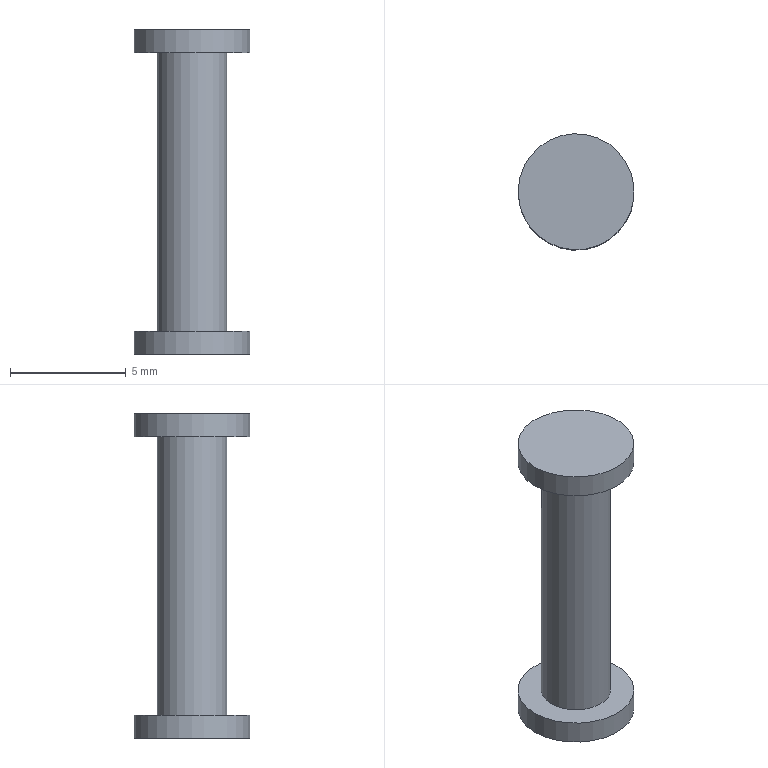Component | NX | PIN | 1 solid | 7 faces | box 5 x 5 x 14 mm | volume 124 mm3 | plane 4 | cylinder 3 | commonest cylinder face diameters 5 x2 3 x1
STEP:
#1=CARTESIAN_POINT('',(0.,0.,0.));
#2=DIRECTION('',(0.,0.,1.));
#3=DIRECTION('',(1.,0.,0.));
#4=AXIS2_PLACEMENT_3D('',#1,#2,#3);
#5=CARTESIAN_POINT('',(-11.268,-58.059,25.35));
#6=VERTEX_POINT('',#5);
#7=CARTESIAN_POINT('',(-9.005,-59.121,25.35));
#8=DIRECTION('',(0.,0.,1.));
#9=DIRECTION('',(-0.9054,0.4247,0.));
#10=AXIS2_PLACEMENT_3D('',#7,#8,#9);
#11=CIRCLE('',#10,2.5);
#12=CARTESIAN_POINT('',(-11.268,-58.059,25.35));
#13=DIRECTION('',(0.,0.,-1.));
#14=DIRECTION('',(0.9054,-0.4247,0.));
#15=AXIS2_PLACEMENT_3D('',#12,#13,#14);
#16=PLANE('',#15);
#17=CARTESIAN_POINT('',(0.,-0.));
#18=CARTESIAN_POINT('',(0.,4.33));
#19=CARTESIAN_POINT('',(3.75,2.165));
#20=CARTESIAN_POINT('',(7.5,-0.));
#21=CARTESIAN_POINT('',(3.75,-2.165));
#22=CARTESIAN_POINT('',(0.,-4.33));
#23=CARTESIAN_POINT('',(0.,-0.));
#24=(BOUNDED_CURVE()B_SPLINE_CURVE(2,(#17,#18,#19,#20,#21,#22,#23),.UNSPECIFIED.,.T.,.F.)B_SPLINE_CURVE_WITH_KNOTS((1,2,2,2,2,1),(-2.094,0.,2.094,4.189,6.283,8.378),.UNSPECIFIED.)CURVE()GEOMETRIC_REPRESENTATION_ITEM()RATIONAL_B_SPLINE_CURVE((1.,0.5,1.,0.5,1.,0.5,1.))REPRESENTATION_ITEM(''));
#25=(GEOMETRIC_REPRESENTATION_CONTEXT(2)PARAMETRIC_REPRESENTATION_CONTEXT()REPRESENTATION_CONTEXT('',''));
#26=DEFINITIONAL_REPRESENTATION('',(#24),#25);
#27=PCURVE('',#16,#26);
#28=CARTESIAN_POINT('',(-9.005,-59.121,25.35));
#29=DIRECTION('',(0.,0.,1.));
#30=DIRECTION('',(-0.9054,0.4247,0.));
#31=AXIS2_PLACEMENT_3D('',#28,#29,#30);
#32=CYLINDRICAL_SURFACE('',#31,2.5);
#33=CARTESIAN_POINT('',(0.,0.));
#34=DIRECTION('',(1.,0.));
#35=VECTOR('',#34,1.);
#36=LINE('',#33,#35);
#37=(GEOMETRIC_REPRESENTATION_CONTEXT(2)PARAMETRIC_REPRESENTATION_CONTEXT()REPRESENTATION_CONTEXT('',''));
#38=DEFINITIONAL_REPRESENTATION('',(#36),#37);
#39=PCURVE('',#32,#38);
#40=SURFACE_CURVE('',#11,(#27,#39),.PCURVE_S1.);
#41=EDGE_CURVE('',#6,#6,#40,.T.);
#42=ORIENTED_EDGE('',*,*,#41,.F.);
#43=EDGE_LOOP('',(#42));
#44=FACE_BOUND('',#43,.T.);
#45=ADVANCED_FACE('',(#44),#16,.T.);
#46=ORIENTED_EDGE('',*,*,#41,.T.);
#47=CARTESIAN_POINT('',(-11.268,-58.059,26.35));
#48=VERTEX_POINT('',#47);
#49=CARTESIAN_POINT('',(-11.268,-58.059,25.35));
#50=CARTESIAN_POINT('',(-11.268,-58.059,26.35));
#51=B_SPLINE_CURVE_WITH_KNOTS('',1,(#49,#50),.UNSPECIFIED.,.F.,.F.,(2,2),(0.,1.),.PIECEWISE_BEZIER_KNOTS.);
#52=CARTESIAN_POINT('',(6.283,0.));
#53=DIRECTION('',(0.,1.));
#54=VECTOR('',#53,1.);
#55=LINE('',#52,#54);
#56=(GEOMETRIC_REPRESENTATION_CONTEXT(2)PARAMETRIC_REPRESENTATION_CONTEXT()REPRESENTATION_CONTEXT('',''));
#57=DEFINITIONAL_REPRESENTATION('',(#55),#56);
#58=PCURVE('',#32,#57);
#59=CARTESIAN_POINT('',(0.,0.));
#60=DIRECTION('',(0.,1.));
#61=VECTOR('',#60,1.);
#62=LINE('',#59,#61);
#63=(GEOMETRIC_REPRESENTATION_CONTEXT(2)PARAMETRIC_REPRESENTATION_CONTEXT()REPRESENTATION_CONTEXT('',''));
#64=DEFINITIONAL_REPRESENTATION('',(#62),#63);
#65=PCURVE('',#32,#64);
#66=SEAM_CURVE('',#51,(#58,#65),.PCURVE_S1.);
#67=EDGE_CURVE('',#6,#48,#66,.T.);
#68=ORIENTED_EDGE('',*,*,#67,.T.);
#69=CARTESIAN_POINT('',(-9.005,-59.121,26.35));
#70=DIRECTION('',(0.,0.,1.));
#71=DIRECTION('',(-0.9054,0.4247,0.));
#72=AXIS2_PLACEMENT_3D('',#69,#70,#71);
#73=CIRCLE('',#72,2.5);
#74=CARTESIAN_POINT('',(0.,1.));
#75=DIRECTION('',(1.,0.));
#76=VECTOR('',#75,1.);
#77=LINE('',#74,#76);
#78=(GEOMETRIC_REPRESENTATION_CONTEXT(2)PARAMETRIC_REPRESENTATION_CONTEXT()REPRESENTATION_CONTEXT('',''));
#79=DEFINITIONAL_REPRESENTATION('',(#77),#78);
#80=PCURVE('',#32,#79);
#81=CARTESIAN_POINT('',(-10.363,-58.484,26.35));
#82=DIRECTION('',(0.,0.,1.));
#83=DIRECTION('',(-0.9054,0.4247,0.));
#84=AXIS2_PLACEMENT_3D('',#81,#82,#83);
#85=PLANE('',#84);
#86=CARTESIAN_POINT('',(-1.5,0.));
#87=DIRECTION('',(1.,0.));
#88=AXIS2_PLACEMENT_2D('',#86,#87);
#89=CIRCLE('',#88,2.5);
#90=(GEOMETRIC_REPRESENTATION_CONTEXT(2)PARAMETRIC_REPRESENTATION_CONTEXT()REPRESENTATION_CONTEXT('',''));
#91=DEFINITIONAL_REPRESENTATION('',(#89),#90);
#92=PCURVE('',#85,#91);
#93=SURFACE_CURVE('',#73,(#80,#92),.PCURVE_S1.);
#94=EDGE_CURVE('',#48,#48,#93,.T.);
#95=ORIENTED_EDGE('',*,*,#94,.F.);
#96=ORIENTED_EDGE('',*,*,#67,.F.);
#97=EDGE_LOOP('',(#46,#68,#95,#96));
#98=FACE_BOUND('',#97,.T.);
#99=ADVANCED_FACE('',(#98),#32,.T.);
#100=ORIENTED_EDGE('',*,*,#94,.T.);
#101=EDGE_LOOP('',(#100));
#102=FACE_BOUND('',#101,.T.);
#103=CARTESIAN_POINT('',(-10.363,-58.484,26.35));
#104=VERTEX_POINT('',#103);
#105=CARTESIAN_POINT('',(-9.005,-59.121,26.35));
#106=DIRECTION('',(0.,0.,1.));
#107=DIRECTION('',(-0.9054,0.4247,0.));
#108=AXIS2_PLACEMENT_3D('',#105,#106,#107);
#109=CIRCLE('',#108,1.5);
#110=CARTESIAN_POINT('',(-1.5,0.));
#111=DIRECTION('',(1.,0.));
#112=AXIS2_PLACEMENT_2D('',#110,#111);
#113=CIRCLE('',#112,1.5);
#114=(GEOMETRIC_REPRESENTATION_CONTEXT(2)PARAMETRIC_REPRESENTATION_CONTEXT()REPRESENTATION_CONTEXT('',''));
#115=DEFINITIONAL_REPRESENTATION('',(#113),#114);
#116=PCURVE('',#85,#115);
#117=CARTESIAN_POINT('',(-9.005,-59.121,25.35));
#118=DIRECTION('',(0.,0.,1.));
#119=DIRECTION('',(-0.9054,0.4247,0.));
#120=AXIS2_PLACEMENT_3D('',#117,#118,#119);
#121=CYLINDRICAL_SURFACE('',#120,1.5);
#122=CARTESIAN_POINT('',(0.,1.));
#123=DIRECTION('',(1.,0.));
#124=VECTOR('',#123,1.);
#125=LINE('',#122,#124);
#126=(GEOMETRIC_REPRESENTATION_CONTEXT(2)PARAMETRIC_REPRESENTATION_CONTEXT()REPRESENTATION_CONTEXT('',''));
#127=DEFINITIONAL_REPRESENTATION('',(#125),#126);
#128=PCURVE('',#121,#127);
#129=SURFACE_CURVE('',#109,(#116,#128),.PCURVE_S1.);
#130=EDGE_CURVE('',#104,#104,#129,.T.);
#131=ORIENTED_EDGE('',*,*,#130,.F.);
#132=EDGE_LOOP('',(#131));
#133=FACE_BOUND('',#132,.T.);
#134=ADVANCED_FACE('',(#102,#133),#85,.T.);
#135=ORIENTED_EDGE('',*,*,#130,.T.);
#136=CARTESIAN_POINT('',(-10.363,-58.484,38.35));
#137=VERTEX_POINT('',#136);
#138=CARTESIAN_POINT('',(-10.363,-58.484,26.35));
#139=CARTESIAN_POINT('',(-10.363,-58.484,38.35));
#140=B_SPLINE_CURVE_WITH_KNOTS('',1,(#138,#139),.UNSPECIFIED.,.F.,.F.,(2,2),(1.,13.),.PIECEWISE_BEZIER_KNOTS.);
#141=CARTESIAN_POINT('',(6.283,0.));
#142=DIRECTION('',(0.,1.));
#143=VECTOR('',#142,1.);
#144=LINE('',#141,#143);
#145=(GEOMETRIC_REPRESENTATION_CONTEXT(2)PARAMETRIC_REPRESENTATION_CONTEXT()REPRESENTATION_CONTEXT('',''));
#146=DEFINITIONAL_REPRESENTATION('',(#144),#145);
#147=PCURVE('',#121,#146);
#148=CARTESIAN_POINT('',(0.,0.));
#149=DIRECTION('',(0.,1.));
#150=VECTOR('',#149,1.);
#151=LINE('',#148,#150);
#152=(GEOMETRIC_REPRESENTATION_CONTEXT(2)PARAMETRIC_REPRESENTATION_CONTEXT()REPRESENTATION_CONTEXT('',''));
#153=DEFINITIONAL_REPRESENTATION('',(#151),#152);
#154=PCURVE('',#121,#153);
#155=SEAM_CURVE('',#140,(#147,#154),.PCURVE_S1.);
#156=EDGE_CURVE('',#104,#137,#155,.T.);
#157=ORIENTED_EDGE('',*,*,#156,.T.);
#158=CARTESIAN_POINT('',(-9.005,-59.121,38.35));
#159=DIRECTION('',(0.,0.,1.));
#160=DIRECTION('',(-0.9054,0.4247,0.));
#161=AXIS2_PLACEMENT_3D('',#158,#159,#160);
#162=CIRCLE('',#161,1.5);
#163=CARTESIAN_POINT('',(0.,13.));
#164=DIRECTION('',(1.,0.));
#165=VECTOR('',#164,1.);
#166=LINE('',#163,#165);
#167=(GEOMETRIC_REPRESENTATION_CONTEXT(2)PARAMETRIC_REPRESENTATION_CONTEXT()REPRESENTATION_CONTEXT('',''));
#168=DEFINITIONAL_REPRESENTATION('',(#166),#167);
#169=PCURVE('',#121,#168);
#170=CARTESIAN_POINT('',(-11.268,-58.059,38.35));
#171=DIRECTION('',(0.,0.,-1.));
#172=DIRECTION('',(0.9054,-0.4247,0.));
#173=AXIS2_PLACEMENT_3D('',#170,#171,#172);
#174=PLANE('',#173);
#175=CARTESIAN_POINT('',(1.,-0.));
#176=CARTESIAN_POINT('',(1.,2.598));
#177=CARTESIAN_POINT('',(3.25,1.299));
#178=CARTESIAN_POINT('',(5.5,-0.));
#179=CARTESIAN_POINT('',(3.25,-1.299));
#180=CARTESIAN_POINT('',(1.,-2.598));
#181=CARTESIAN_POINT('',(1.,-0.));
#182=(BOUNDED_CURVE()B_SPLINE_CURVE(2,(#175,#176,#177,#178,#179,#180,#181),.UNSPECIFIED.,.T.,.F.)B_SPLINE_CURVE_WITH_KNOTS((1,2,2,2,2,1),(-2.094,0.,2.094,4.189,6.283,8.378),.UNSPECIFIED.)CURVE()GEOMETRIC_REPRESENTATION_ITEM()RATIONAL_B_SPLINE_CURVE((1.,0.5,1.,0.5,1.,0.5,1.))REPRESENTATION_ITEM(''));
#183=(GEOMETRIC_REPRESENTATION_CONTEXT(2)PARAMETRIC_REPRESENTATION_CONTEXT()REPRESENTATION_CONTEXT('',''));
#184=DEFINITIONAL_REPRESENTATION('',(#182),#183);
#185=PCURVE('',#174,#184);
#186=SURFACE_CURVE('',#162,(#169,#185),.PCURVE_S1.);
#187=EDGE_CURVE('',#137,#137,#186,.T.);
#188=ORIENTED_EDGE('',*,*,#187,.F.);
#189=ORIENTED_EDGE('',*,*,#156,.F.);
#190=EDGE_LOOP('',(#135,#157,#188,#189));
#191=FACE_BOUND('',#190,.T.);
#192=ADVANCED_FACE('',(#191),#121,.T.);
#193=ORIENTED_EDGE('',*,*,#187,.T.);
#194=EDGE_LOOP('',(#193));
#195=FACE_BOUND('',#194,.T.);
#196=CARTESIAN_POINT('',(-11.268,-58.059,38.35));
#197=VERTEX_POINT('',#196);
#198=CARTESIAN_POINT('',(-9.005,-59.121,38.35));
#199=DIRECTION('',(0.,0.,1.));
#200=DIRECTION('',(-0.9054,0.4247,0.));
#201=AXIS2_PLACEMENT_3D('',#198,#199,#200);
#202=CIRCLE('',#201,2.5);
#203=CARTESIAN_POINT('',(0.,-0.));
#204=CARTESIAN_POINT('',(0.,4.33));
#205=CARTESIAN_POINT('',(3.75,2.165));
#206=CARTESIAN_POINT('',(7.5,-0.));
#207=CARTESIAN_POINT('',(3.75,-2.165));
#208=CARTESIAN_POINT('',(0.,-4.33));
#209=CARTESIAN_POINT('',(0.,-0.));
#210=(BOUNDED_CURVE()B_SPLINE_CURVE(2,(#203,#204,#205,#206,#207,#208,#209),.UNSPECIFIED.,.T.,.F.)B_SPLINE_CURVE_WITH_KNOTS((1,2,2,2,2,1),(-2.094,0.,2.094,4.189,6.283,8.378),.UNSPECIFIED.)CURVE()GEOMETRIC_REPRESENTATION_ITEM()RATIONAL_B_SPLINE_CURVE((1.,0.5,1.,0.5,1.,0.5,1.))REPRESENTATION_ITEM(''));
#211=(GEOMETRIC_REPRESENTATION_CONTEXT(2)PARAMETRIC_REPRESENTATION_CONTEXT()REPRESENTATION_CONTEXT('',''));
#212=DEFINITIONAL_REPRESENTATION('',(#210),#211);
#213=PCURVE('',#174,#212);
#214=CARTESIAN_POINT('',(-9.005,-59.121,25.35));
#215=DIRECTION('',(0.,0.,1.));
#216=DIRECTION('',(-0.9054,0.4247,0.));
#217=AXIS2_PLACEMENT_3D('',#214,#215,#216);
#218=CYLINDRICAL_SURFACE('',#217,2.5);
#219=CARTESIAN_POINT('',(0.,13.));
#220=DIRECTION('',(1.,0.));
#221=VECTOR('',#220,1.);
#222=LINE('',#219,#221);
#223=(GEOMETRIC_REPRESENTATION_CONTEXT(2)PARAMETRIC_REPRESENTATION_CONTEXT()REPRESENTATION_CONTEXT('',''));
#224=DEFINITIONAL_REPRESENTATION('',(#222),#223);
#225=PCURVE('',#218,#224);
#226=SURFACE_CURVE('',#202,(#213,#225),.PCURVE_S1.);
#227=EDGE_CURVE('',#197,#197,#226,.T.);
#228=ORIENTED_EDGE('',*,*,#227,.F.);
#229=EDGE_LOOP('',(#228));
#230=FACE_BOUND('',#229,.T.);
#231=ADVANCED_FACE('',(#195,#230),#174,.T.);
#232=ORIENTED_EDGE('',*,*,#227,.T.);
#233=CARTESIAN_POINT('',(-11.268,-58.059,39.35));
#234=VERTEX_POINT('',#233);
#235=CARTESIAN_POINT('',(-11.268,-58.059,38.35));
#236=CARTESIAN_POINT('',(-11.268,-58.059,39.35));
#237=B_SPLINE_CURVE_WITH_KNOTS('',1,(#235,#236),.UNSPECIFIED.,.F.,.F.,(2,2),(13.,14.),.PIECEWISE_BEZIER_KNOTS.);
#238=CARTESIAN_POINT('',(6.283,0.));
#239=DIRECTION('',(0.,1.));
#240=VECTOR('',#239,1.);
#241=LINE('',#238,#240);
#242=(GEOMETRIC_REPRESENTATION_CONTEXT(2)PARAMETRIC_REPRESENTATION_CONTEXT()REPRESENTATION_CONTEXT('',''));
#243=DEFINITIONAL_REPRESENTATION('',(#241),#242);
#244=PCURVE('',#218,#243);
#245=CARTESIAN_POINT('',(0.,0.));
#246=DIRECTION('',(0.,1.));
#247=VECTOR('',#246,1.);
#248=LINE('',#245,#247);
#249=(GEOMETRIC_REPRESENTATION_CONTEXT(2)PARAMETRIC_REPRESENTATION_CONTEXT()REPRESENTATION_CONTEXT('',''));
#250=DEFINITIONAL_REPRESENTATION('',(#248),#249);
#251=PCURVE('',#218,#250);
#252=SEAM_CURVE('',#237,(#244,#251),.PCURVE_S1.);
#253=EDGE_CURVE('',#197,#234,#252,.T.);
#254=ORIENTED_EDGE('',*,*,#253,.T.);
#255=CARTESIAN_POINT('',(-9.005,-59.121,39.35));
#256=DIRECTION('',(0.,0.,1.));
#257=DIRECTION('',(-0.9054,0.4247,0.));
#258=AXIS2_PLACEMENT_3D('',#255,#256,#257);
#259=CIRCLE('',#258,2.5);
#260=CARTESIAN_POINT('',(0.,14.));
#261=DIRECTION('',(1.,0.));
#262=VECTOR('',#261,1.);
#263=LINE('',#260,#262);
#264=(GEOMETRIC_REPRESENTATION_CONTEXT(2)PARAMETRIC_REPRESENTATION_CONTEXT()REPRESENTATION_CONTEXT('',''));
#265=DEFINITIONAL_REPRESENTATION('',(#263),#264);
#266=PCURVE('',#218,#265);
#267=CARTESIAN_POINT('',(-9.005,-59.121,39.35));
#268=DIRECTION('',(0.,0.,1.));
#269=DIRECTION('',(-0.9054,0.4247,0.));
#270=AXIS2_PLACEMENT_3D('',#267,#268,#269);
#271=PLANE('',#270);
#272=CARTESIAN_POINT('',(0.,0.));
#273=DIRECTION('',(1.,0.));
#274=AXIS2_PLACEMENT_2D('',#272,#273);
#275=CIRCLE('',#274,2.5);
#276=(GEOMETRIC_REPRESENTATION_CONTEXT(2)PARAMETRIC_REPRESENTATION_CONTEXT()REPRESENTATION_CONTEXT('',''));
#277=DEFINITIONAL_REPRESENTATION('',(#275),#276);
#278=PCURVE('',#271,#277);
#279=SURFACE_CURVE('',#259,(#266,#278),.PCURVE_S1.);
#280=EDGE_CURVE('',#234,#234,#279,.T.);
#281=ORIENTED_EDGE('',*,*,#280,.F.);
#282=ORIENTED_EDGE('',*,*,#253,.F.);
#283=EDGE_LOOP('',(#232,#254,#281,#282));
#284=FACE_BOUND('',#283,.T.);
#285=ADVANCED_FACE('',(#284),#218,.T.);
#286=ORIENTED_EDGE('',*,*,#280,.T.);
#287=EDGE_LOOP('',(#286));
#288=FACE_BOUND('',#287,.T.);
#289=ADVANCED_FACE('',(#288),#271,.T.);
#290=CLOSED_SHELL('',(#45,#99,#134,#192,#231,#285,#289));
#291=MANIFOLD_SOLID_BREP('',#290);
#292=(LENGTH_UNIT()NAMED_UNIT(*)SI_UNIT(.MILLI.,.METRE.));
#293=UNCERTAINTY_MEASURE_WITH_UNIT(LENGTH_MEASURE(0.00001),#292,'','');
#294=(NAMED_UNIT(*)PLANE_ANGLE_UNIT()SI_UNIT($,.RADIAN.));
#295=(NAMED_UNIT(*)SI_UNIT($,.STERADIAN.)SOLID_ANGLE_UNIT());
#296=(GEOMETRIC_REPRESENTATION_CONTEXT(3)GLOBAL_UNCERTAINTY_ASSIGNED_CONTEXT((#293))GLOBAL_UNIT_ASSIGNED_CONTEXT((#292,#294,#295))REPRESENTATION_CONTEXT('',''));
#297=ADVANCED_BREP_SHAPE_REPRESENTATION('',(#4,#291),#296);